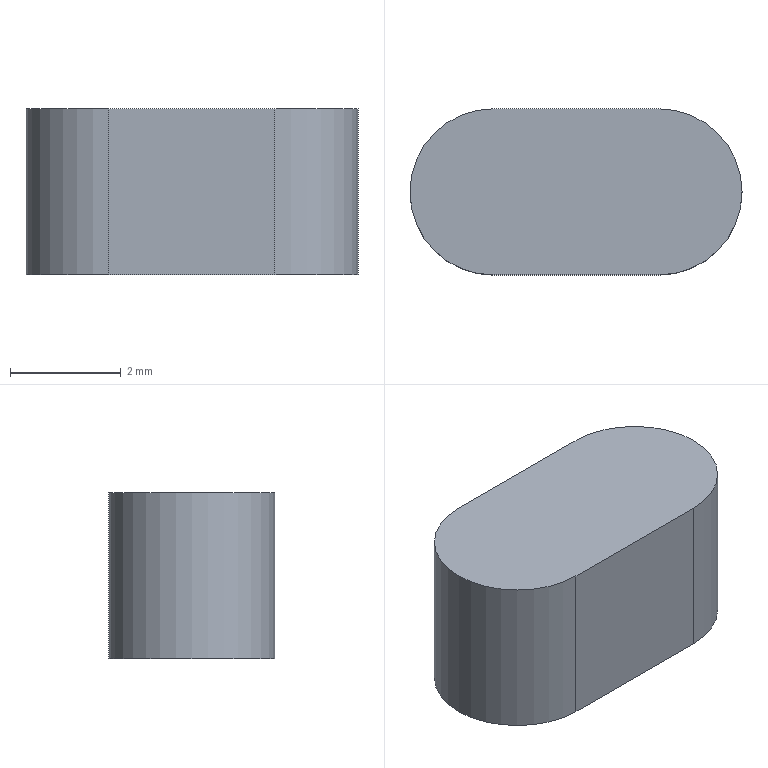Component | NX | ASSY_PRAC_PART_6 | 1 solid | 6 faces | box 6 x 3 x 3 mm | volume 48 mm3 | plane 4 | cylinder 2 | commonest cylinder face diameters 3 x2
STEP:
#1=CARTESIAN_POINT('',(0.,0.,0.));
#2=DIRECTION('',(0.,0.,1.));
#3=DIRECTION('',(1.,0.,0.));
#4=AXIS2_PLACEMENT_3D('',#1,#2,#3);
#5=CARTESIAN_POINT('',(5.76,1.885,22.561));
#6=VERTEX_POINT('',#5);
#7=CARTESIAN_POINT('',(5.76,-1.115,22.561));
#8=VERTEX_POINT('',#7);
#9=CARTESIAN_POINT('',(5.76,0.3851,22.561));
#10=DIRECTION('',(0.,0.,1.));
#11=DIRECTION('',(1.,0.,0.));
#12=AXIS2_PLACEMENT_3D('',#9,#10,#11);
#13=CIRCLE('',#12,1.5);
#14=CARTESIAN_POINT('',(5.76,0.3851,25.561));
#15=DIRECTION('',(0.,0.,-1.));
#16=DIRECTION('',(-1.,0.,0.));
#17=AXIS2_PLACEMENT_3D('',#14,#15,#16);
#18=CYLINDRICAL_SURFACE('',#17,1.5);
#19=CARTESIAN_POINT('',(3.142,3.));
#20=DIRECTION('',(-1.,0.));
#21=VECTOR('',#20,1.);
#22=LINE('',#19,#21);
#23=(GEOMETRIC_REPRESENTATION_CONTEXT(2)PARAMETRIC_REPRESENTATION_CONTEXT()REPRESENTATION_CONTEXT('',''));
#24=DEFINITIONAL_REPRESENTATION('',(#22),#23);
#25=PCURVE('',#18,#24);
#26=CARTESIAN_POINT('',(5.76,0.3851,22.561));
#27=DIRECTION('',(0.,0.,1.));
#28=DIRECTION('',(1.,0.,0.));
#29=AXIS2_PLACEMENT_3D('',#26,#27,#28);
#30=PLANE('',#29);
#31=CARTESIAN_POINT('',(0.,0.));
#32=DIRECTION('',(1.,0.));
#33=AXIS2_PLACEMENT_2D('',#31,#32);
#34=CIRCLE('',#33,1.5);
#35=(GEOMETRIC_REPRESENTATION_CONTEXT(2)PARAMETRIC_REPRESENTATION_CONTEXT()REPRESENTATION_CONTEXT('',''));
#36=DEFINITIONAL_REPRESENTATION('',(#34),#35);
#37=PCURVE('',#30,#36);
#38=SURFACE_CURVE('',#13,(#25,#37),.PCURVE_S1.);
#39=EDGE_CURVE('',#6,#8,#38,.T.);
#40=ORIENTED_EDGE('',*,*,#39,.T.);
#41=CARTESIAN_POINT('',(5.76,-1.115,25.561));
#42=VERTEX_POINT('',#41);
#43=CARTESIAN_POINT('',(5.76,-1.115,25.561));
#44=DIRECTION('',(0.,0.,-1.));
#45=VECTOR('',#44,1.);
#46=LINE('',#43,#45);
#47=CARTESIAN_POINT('',(-1.571,0.));
#48=DIRECTION('',(0.,1.));
#49=VECTOR('',#48,1.);
#50=LINE('',#47,#49);
#51=(GEOMETRIC_REPRESENTATION_CONTEXT(2)PARAMETRIC_REPRESENTATION_CONTEXT()REPRESENTATION_CONTEXT('',''));
#52=DEFINITIONAL_REPRESENTATION('',(#50),#51);
#53=PCURVE('',#18,#52);
#54=CARTESIAN_POINT('',(5.76,-1.115,25.561));
#55=DIRECTION('',(0.,1.,0.));
#56=DIRECTION('',(0.,0.,1.));
#57=AXIS2_PLACEMENT_3D('',#54,#55,#56);
#58=PLANE('',#57);
#59=CARTESIAN_POINT('',(0.,0.));
#60=DIRECTION('',(-1.,0.));
#61=VECTOR('',#60,1.);
#62=LINE('',#59,#61);
#63=(GEOMETRIC_REPRESENTATION_CONTEXT(2)PARAMETRIC_REPRESENTATION_CONTEXT()REPRESENTATION_CONTEXT('',''));
#64=DEFINITIONAL_REPRESENTATION('',(#62),#63);
#65=PCURVE('',#58,#64);
#66=SURFACE_CURVE('',#46,(#53,#65),.PCURVE_S1.);
#67=EDGE_CURVE('',#42,#8,#66,.T.);
#68=ORIENTED_EDGE('',*,*,#67,.F.);
#69=CARTESIAN_POINT('',(5.76,1.885,25.561));
#70=VERTEX_POINT('',#69);
#71=CARTESIAN_POINT('',(5.76,0.3851,25.561));
#72=DIRECTION('',(0.,0.,1.));
#73=DIRECTION('',(1.,0.,0.));
#74=AXIS2_PLACEMENT_3D('',#71,#72,#73);
#75=CIRCLE('',#74,1.5);
#76=CARTESIAN_POINT('',(3.142,0.));
#77=DIRECTION('',(-1.,0.));
#78=VECTOR('',#77,1.);
#79=LINE('',#76,#78);
#80=(GEOMETRIC_REPRESENTATION_CONTEXT(2)PARAMETRIC_REPRESENTATION_CONTEXT()REPRESENTATION_CONTEXT('',''));
#81=DEFINITIONAL_REPRESENTATION('',(#79),#80);
#82=PCURVE('',#18,#81);
#83=CARTESIAN_POINT('',(5.76,0.3851,25.561));
#84=DIRECTION('',(0.,0.,1.));
#85=DIRECTION('',(1.,0.,0.));
#86=AXIS2_PLACEMENT_3D('',#83,#84,#85);
#87=PLANE('',#86);
#88=CARTESIAN_POINT('',(0.,0.));
#89=DIRECTION('',(1.,0.));
#90=AXIS2_PLACEMENT_2D('',#88,#89);
#91=CIRCLE('',#90,1.5);
#92=(GEOMETRIC_REPRESENTATION_CONTEXT(2)PARAMETRIC_REPRESENTATION_CONTEXT()REPRESENTATION_CONTEXT('',''));
#93=DEFINITIONAL_REPRESENTATION('',(#91),#92);
#94=PCURVE('',#87,#93);
#95=SURFACE_CURVE('',#75,(#82,#94),.PCURVE_S1.);
#96=EDGE_CURVE('',#70,#42,#95,.T.);
#97=ORIENTED_EDGE('',*,*,#96,.F.);
#98=CARTESIAN_POINT('',(5.76,1.885,25.561));
#99=DIRECTION('',(0.,0.,-1.));
#100=VECTOR('',#99,1.);
#101=LINE('',#98,#100);
#102=CARTESIAN_POINT('',(1.571,0.));
#103=DIRECTION('',(0.,1.));
#104=VECTOR('',#103,1.);
#105=LINE('',#102,#104);
#106=(GEOMETRIC_REPRESENTATION_CONTEXT(2)PARAMETRIC_REPRESENTATION_CONTEXT()REPRESENTATION_CONTEXT('',''));
#107=DEFINITIONAL_REPRESENTATION('',(#105),#106);
#108=PCURVE('',#18,#107);
#109=CARTESIAN_POINT('',(8.76,1.885,25.561));
#110=DIRECTION('',(0.,-1.,0.));
#111=DIRECTION('',(0.,0.,-1.));
#112=AXIS2_PLACEMENT_3D('',#109,#110,#111);
#113=PLANE('',#112);
#114=CARTESIAN_POINT('',(0.,-3.));
#115=DIRECTION('',(1.,0.));
#116=VECTOR('',#115,1.);
#117=LINE('',#114,#116);
#118=(GEOMETRIC_REPRESENTATION_CONTEXT(2)PARAMETRIC_REPRESENTATION_CONTEXT()REPRESENTATION_CONTEXT('',''));
#119=DEFINITIONAL_REPRESENTATION('',(#117),#118);
#120=PCURVE('',#113,#119);
#121=SURFACE_CURVE('',#101,(#108,#120),.PCURVE_S1.);
#122=EDGE_CURVE('',#70,#6,#121,.T.);
#123=ORIENTED_EDGE('',*,*,#122,.T.);
#124=EDGE_LOOP('',(#40,#68,#97,#123));
#125=FACE_BOUND('',#124,.T.);
#126=ADVANCED_FACE('',(#125),#18,.T.);
#127=CARTESIAN_POINT('',(8.76,-1.115,22.561));
#128=VERTEX_POINT('',#127);
#129=CARTESIAN_POINT('',(5.76,-1.115,22.561));
#130=DIRECTION('',(1.,0.,0.));
#131=VECTOR('',#130,1.);
#132=LINE('',#129,#131);
#133=CARTESIAN_POINT('',(-3.,0.));
#134=DIRECTION('',(0.,1.));
#135=VECTOR('',#134,1.);
#136=LINE('',#133,#135);
#137=(GEOMETRIC_REPRESENTATION_CONTEXT(2)PARAMETRIC_REPRESENTATION_CONTEXT()REPRESENTATION_CONTEXT('',''));
#138=DEFINITIONAL_REPRESENTATION('',(#136),#137);
#139=PCURVE('',#58,#138);
#140=CARTESIAN_POINT('',(0.,-1.5));
#141=DIRECTION('',(1.,0.));
#142=VECTOR('',#141,1.);
#143=LINE('',#140,#142);
#144=(GEOMETRIC_REPRESENTATION_CONTEXT(2)PARAMETRIC_REPRESENTATION_CONTEXT()REPRESENTATION_CONTEXT('',''));
#145=DEFINITIONAL_REPRESENTATION('',(#143),#144);
#146=PCURVE('',#30,#145);
#147=SURFACE_CURVE('',#132,(#139,#146),.PCURVE_S1.);
#148=EDGE_CURVE('',#8,#128,#147,.T.);
#149=ORIENTED_EDGE('',*,*,#148,.T.);
#150=CARTESIAN_POINT('',(8.76,-1.115,25.561));
#151=VERTEX_POINT('',#150);
#152=CARTESIAN_POINT('',(8.76,-1.115,25.561));
#153=DIRECTION('',(0.,0.,-1.));
#154=VECTOR('',#153,1.);
#155=LINE('',#152,#154);
#156=CARTESIAN_POINT('',(0.,3.));
#157=DIRECTION('',(-1.,0.));
#158=VECTOR('',#157,1.);
#159=LINE('',#156,#158);
#160=(GEOMETRIC_REPRESENTATION_CONTEXT(2)PARAMETRIC_REPRESENTATION_CONTEXT()REPRESENTATION_CONTEXT('',''));
#161=DEFINITIONAL_REPRESENTATION('',(#159),#160);
#162=PCURVE('',#58,#161);
#163=CARTESIAN_POINT('',(8.76,0.3851,25.561));
#164=DIRECTION('',(0.,0.,-1.));
#165=DIRECTION('',(-1.,0.,0.));
#166=AXIS2_PLACEMENT_3D('',#163,#164,#165);
#167=CYLINDRICAL_SURFACE('',#166,1.5);
#168=CARTESIAN_POINT('',(4.712,0.));
#169=DIRECTION('',(0.,1.));
#170=VECTOR('',#169,1.);
#171=LINE('',#168,#170);
#172=(GEOMETRIC_REPRESENTATION_CONTEXT(2)PARAMETRIC_REPRESENTATION_CONTEXT()REPRESENTATION_CONTEXT('',''));
#173=DEFINITIONAL_REPRESENTATION('',(#171),#172);
#174=PCURVE('',#167,#173);
#175=SURFACE_CURVE('',#155,(#162,#174),.PCURVE_S1.);
#176=EDGE_CURVE('',#151,#128,#175,.T.);
#177=ORIENTED_EDGE('',*,*,#176,.F.);
#178=CARTESIAN_POINT('',(5.76,-1.115,25.561));
#179=DIRECTION('',(1.,0.,0.));
#180=VECTOR('',#179,1.);
#181=LINE('',#178,#180);
#182=CARTESIAN_POINT('',(0.,0.));
#183=DIRECTION('',(0.,1.));
#184=VECTOR('',#183,1.);
#185=LINE('',#182,#184);
#186=(GEOMETRIC_REPRESENTATION_CONTEXT(2)PARAMETRIC_REPRESENTATION_CONTEXT()REPRESENTATION_CONTEXT('',''));
#187=DEFINITIONAL_REPRESENTATION('',(#185),#186);
#188=PCURVE('',#58,#187);
#189=CARTESIAN_POINT('',(0.,-1.5));
#190=DIRECTION('',(1.,0.));
#191=VECTOR('',#190,1.);
#192=LINE('',#189,#191);
#193=(GEOMETRIC_REPRESENTATION_CONTEXT(2)PARAMETRIC_REPRESENTATION_CONTEXT()REPRESENTATION_CONTEXT('',''));
#194=DEFINITIONAL_REPRESENTATION('',(#192),#193);
#195=PCURVE('',#87,#194);
#196=SURFACE_CURVE('',#181,(#188,#195),.PCURVE_S1.);
#197=EDGE_CURVE('',#42,#151,#196,.T.);
#198=ORIENTED_EDGE('',*,*,#197,.F.);
#199=ORIENTED_EDGE('',*,*,#67,.T.);
#200=EDGE_LOOP('',(#149,#177,#198,#199));
#201=FACE_BOUND('',#200,.T.);
#202=ADVANCED_FACE('',(#201),#58,.F.);
#203=CARTESIAN_POINT('',(8.76,1.885,22.561));
#204=VERTEX_POINT('',#203);
#205=CARTESIAN_POINT('',(8.76,0.3851,22.561));
#206=DIRECTION('',(0.,0.,1.));
#207=DIRECTION('',(1.,0.,0.));
#208=AXIS2_PLACEMENT_3D('',#205,#206,#207);
#209=CIRCLE('',#208,1.5);
#210=CARTESIAN_POINT('',(9.425,3.));
#211=DIRECTION('',(-1.,0.));
#212=VECTOR('',#211,1.);
#213=LINE('',#210,#212);
#214=(GEOMETRIC_REPRESENTATION_CONTEXT(2)PARAMETRIC_REPRESENTATION_CONTEXT()REPRESENTATION_CONTEXT('',''));
#215=DEFINITIONAL_REPRESENTATION('',(#213),#214);
#216=PCURVE('',#167,#215);
#217=CARTESIAN_POINT('',(3.,0.));
#218=DIRECTION('',(1.,0.));
#219=AXIS2_PLACEMENT_2D('',#217,#218);
#220=CIRCLE('',#219,1.5);
#221=(GEOMETRIC_REPRESENTATION_CONTEXT(2)PARAMETRIC_REPRESENTATION_CONTEXT()REPRESENTATION_CONTEXT('',''));
#222=DEFINITIONAL_REPRESENTATION('',(#220),#221);
#223=PCURVE('',#30,#222);
#224=SURFACE_CURVE('',#209,(#216,#223),.PCURVE_S1.);
#225=EDGE_CURVE('',#128,#204,#224,.T.);
#226=ORIENTED_EDGE('',*,*,#225,.T.);
#227=CARTESIAN_POINT('',(8.76,1.885,25.561));
#228=VERTEX_POINT('',#227);
#229=CARTESIAN_POINT('',(8.76,1.885,25.561));
#230=DIRECTION('',(0.,0.,-1.));
#231=VECTOR('',#230,1.);
#232=LINE('',#229,#231);
#233=CARTESIAN_POINT('',(1.571,0.));
#234=DIRECTION('',(0.,1.));
#235=VECTOR('',#234,1.);
#236=LINE('',#233,#235);
#237=(GEOMETRIC_REPRESENTATION_CONTEXT(2)PARAMETRIC_REPRESENTATION_CONTEXT()REPRESENTATION_CONTEXT('',''));
#238=DEFINITIONAL_REPRESENTATION('',(#236),#237);
#239=PCURVE('',#167,#238);
#240=CARTESIAN_POINT('',(0.,0.));
#241=DIRECTION('',(1.,0.));
#242=VECTOR('',#241,1.);
#243=LINE('',#240,#242);
#244=(GEOMETRIC_REPRESENTATION_CONTEXT(2)PARAMETRIC_REPRESENTATION_CONTEXT()REPRESENTATION_CONTEXT('',''));
#245=DEFINITIONAL_REPRESENTATION('',(#243),#244);
#246=PCURVE('',#113,#245);
#247=SURFACE_CURVE('',#232,(#239,#246),.PCURVE_S1.);
#248=EDGE_CURVE('',#228,#204,#247,.T.);
#249=ORIENTED_EDGE('',*,*,#248,.F.);
#250=CARTESIAN_POINT('',(8.76,0.3851,25.561));
#251=DIRECTION('',(0.,0.,1.));
#252=DIRECTION('',(1.,0.,0.));
#253=AXIS2_PLACEMENT_3D('',#250,#251,#252);
#254=CIRCLE('',#253,1.5);
#255=CARTESIAN_POINT('',(9.425,0.));
#256=DIRECTION('',(-1.,0.));
#257=VECTOR('',#256,1.);
#258=LINE('',#255,#257);
#259=(GEOMETRIC_REPRESENTATION_CONTEXT(2)PARAMETRIC_REPRESENTATION_CONTEXT()REPRESENTATION_CONTEXT('',''));
#260=DEFINITIONAL_REPRESENTATION('',(#258),#259);
#261=PCURVE('',#167,#260);
#262=CARTESIAN_POINT('',(3.,0.));
#263=DIRECTION('',(1.,0.));
#264=AXIS2_PLACEMENT_2D('',#262,#263);
#265=CIRCLE('',#264,1.5);
#266=(GEOMETRIC_REPRESENTATION_CONTEXT(2)PARAMETRIC_REPRESENTATION_CONTEXT()REPRESENTATION_CONTEXT('',''));
#267=DEFINITIONAL_REPRESENTATION('',(#265),#266);
#268=PCURVE('',#87,#267);
#269=SURFACE_CURVE('',#254,(#261,#268),.PCURVE_S1.);
#270=EDGE_CURVE('',#151,#228,#269,.T.);
#271=ORIENTED_EDGE('',*,*,#270,.F.);
#272=ORIENTED_EDGE('',*,*,#176,.T.);
#273=EDGE_LOOP('',(#226,#249,#271,#272));
#274=FACE_BOUND('',#273,.T.);
#275=ADVANCED_FACE('',(#274),#167,.T.);
#276=CARTESIAN_POINT('',(8.76,1.885,22.561));
#277=DIRECTION('',(-1.,0.,0.));
#278=VECTOR('',#277,1.);
#279=LINE('',#276,#278);
#280=CARTESIAN_POINT('',(3.,0.));
#281=DIRECTION('',(0.,-1.));
#282=VECTOR('',#281,1.);
#283=LINE('',#280,#282);
#284=(GEOMETRIC_REPRESENTATION_CONTEXT(2)PARAMETRIC_REPRESENTATION_CONTEXT()REPRESENTATION_CONTEXT('',''));
#285=DEFINITIONAL_REPRESENTATION('',(#283),#284);
#286=PCURVE('',#113,#285);
#287=CARTESIAN_POINT('',(3.,1.5));
#288=DIRECTION('',(-1.,0.));
#289=VECTOR('',#288,1.);
#290=LINE('',#287,#289);
#291=(GEOMETRIC_REPRESENTATION_CONTEXT(2)PARAMETRIC_REPRESENTATION_CONTEXT()REPRESENTATION_CONTEXT('',''));
#292=DEFINITIONAL_REPRESENTATION('',(#290),#291);
#293=PCURVE('',#30,#292);
#294=SURFACE_CURVE('',#279,(#286,#293),.PCURVE_S1.);
#295=EDGE_CURVE('',#204,#6,#294,.T.);
#296=ORIENTED_EDGE('',*,*,#295,.T.);
#297=ORIENTED_EDGE('',*,*,#122,.F.);
#298=CARTESIAN_POINT('',(8.76,1.885,25.561));
#299=DIRECTION('',(-1.,0.,0.));
#300=VECTOR('',#299,1.);
#301=LINE('',#298,#300);
#302=CARTESIAN_POINT('',(0.,0.));
#303=DIRECTION('',(0.,-1.));
#304=VECTOR('',#303,1.);
#305=LINE('',#302,#304);
#306=(GEOMETRIC_REPRESENTATION_CONTEXT(2)PARAMETRIC_REPRESENTATION_CONTEXT()REPRESENTATION_CONTEXT('',''));
#307=DEFINITIONAL_REPRESENTATION('',(#305),#306);
#308=PCURVE('',#113,#307);
#309=CARTESIAN_POINT('',(3.,1.5));
#310=DIRECTION('',(-1.,0.));
#311=VECTOR('',#310,1.);
#312=LINE('',#309,#311);
#313=(GEOMETRIC_REPRESENTATION_CONTEXT(2)PARAMETRIC_REPRESENTATION_CONTEXT()REPRESENTATION_CONTEXT('',''));
#314=DEFINITIONAL_REPRESENTATION('',(#312),#313);
#315=PCURVE('',#87,#314);
#316=SURFACE_CURVE('',#301,(#308,#315),.PCURVE_S1.);
#317=EDGE_CURVE('',#228,#70,#316,.T.);
#318=ORIENTED_EDGE('',*,*,#317,.F.);
#319=ORIENTED_EDGE('',*,*,#248,.T.);
#320=EDGE_LOOP('',(#296,#297,#318,#319));
#321=FACE_BOUND('',#320,.T.);
#322=ADVANCED_FACE('',(#321),#113,.F.);
#323=ORIENTED_EDGE('',*,*,#96,.T.);
#324=ORIENTED_EDGE('',*,*,#197,.T.);
#325=ORIENTED_EDGE('',*,*,#270,.T.);
#326=ORIENTED_EDGE('',*,*,#317,.T.);
#327=EDGE_LOOP('',(#323,#324,#325,#326));
#328=FACE_BOUND('',#327,.T.);
#329=ADVANCED_FACE('',(#328),#87,.T.);
#330=ORIENTED_EDGE('',*,*,#39,.F.);
#331=ORIENTED_EDGE('',*,*,#295,.F.);
#332=ORIENTED_EDGE('',*,*,#225,.F.);
#333=ORIENTED_EDGE('',*,*,#148,.F.);
#334=EDGE_LOOP('',(#330,#331,#332,#333));
#335=FACE_BOUND('',#334,.T.);
#336=ADVANCED_FACE('',(#335),#30,.F.);
#337=CLOSED_SHELL('',(#126,#202,#275,#322,#329,#336));
#338=MANIFOLD_SOLID_BREP('',#337);
#339=(LENGTH_UNIT()NAMED_UNIT(*)SI_UNIT(.MILLI.,.METRE.));
#340=UNCERTAINTY_MEASURE_WITH_UNIT(LENGTH_MEASURE(0.0000001),#339,'','');
#341=(NAMED_UNIT(*)PLANE_ANGLE_UNIT()SI_UNIT($,.RADIAN.));
#342=(NAMED_UNIT(*)SI_UNIT($,.STERADIAN.)SOLID_ANGLE_UNIT());
#343=(GEOMETRIC_REPRESENTATION_CONTEXT(3)GLOBAL_UNCERTAINTY_ASSIGNED_CONTEXT((#340))GLOBAL_UNIT_ASSIGNED_CONTEXT((#339,#341,#342))REPRESENTATION_CONTEXT('',''));
#344=ADVANCED_BREP_SHAPE_REPRESENTATION('',(#4,#338),#343);